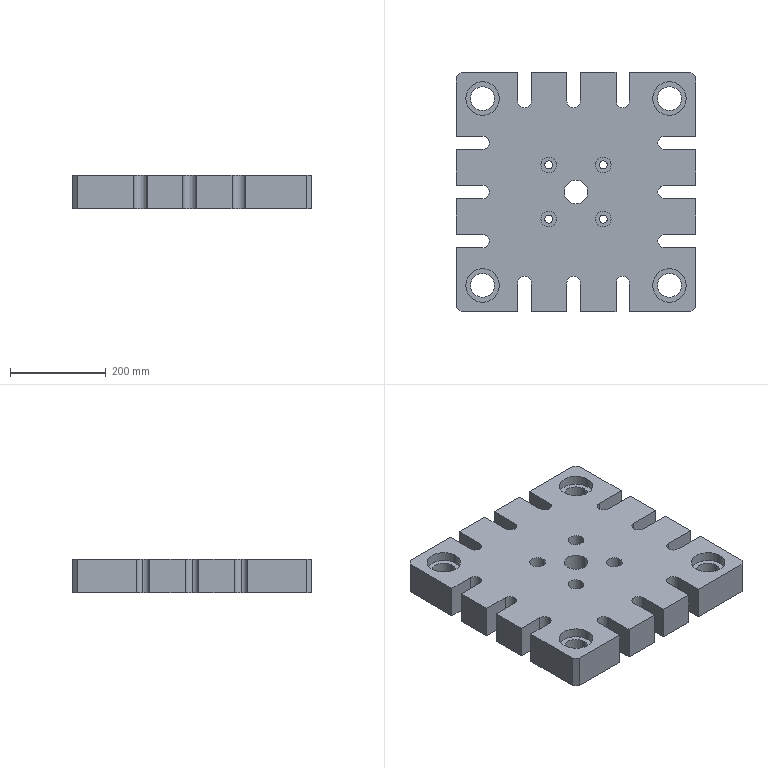Component | SolidWorks | LowerDiePlate-1 | 1 solid | 106 faces | box 500 x 500 x 70 mm | volume 14696489 mm3 | plane 55 | cylinder 51 | commonest cylinder face diameters 28 x15 50 x10 33 x8 70 x8 17 x8 200 x2
build123d program:
from build123d import *

# Parameters (mm, degrees)
SKETCH2_W               = 500
SKETCH2_H               = 500
SKETCH2_R               = 25
BOSS_EXTRUDE1_DEPTH     = 70
SKETCH3_R               = 25
CUT_EXTRUDE1_DEPTH      = 361.416
CUT_EXTRUDE2_DEPTH      = 361.416
CHAMFER1_SIZE           = 10
SKETCH5_R               = 35
CUT_EXTRUDE3_DEPTH      = 20
SKETCH6_R               = 100
CUT_EXTRUDE4_DEPTH      = 5
CUT_EXTRUDE5_DEPTH      = 360.479
CUT_EXTRUDE5_DEPTH_BACK = 360.479
SKETCH7_R               = 8.5
SKETCH8_R               = 16.5
CUT_EXTRUDE6_DEPTH      = 30


with BuildPart() as part:
    # Sketch2 → Boss-Extrude1 (new body)
    with BuildSketch(Plane.XY):
        Rectangle(SKETCH2_W, SKETCH2_H)
        Circle(SKETCH2_R, mode=Mode.SUBTRACT)
    extrude(amount=BOSS_EXTRUDE1_DEPTH)

    # Sketch3 → Cut-Extrude1 (cut, through all)
    with BuildSketch(Plane.XY.offset(70)):
        with Locations((-195, 195)):
            Circle(SKETCH3_R)
        with Locations(Location((195, 195, 0), (0, 0, 180))):
            Circle(SKETCH3_R)
        with Locations((195, -195)):
            Circle(SKETCH3_R)
        with Locations(Location((-195, -195, 0), (0, 0, 180))):
            Circle(SKETCH3_R)
    extrude(amount=-CUT_EXTRUDE1_DEPTH, mode=Mode.SUBTRACT)

    # Sketch4 → Cut-Extrude2 (cut, through all)
    with BuildSketch(Plane.XY.offset(70)):
        with BuildLine():
            Line((-195, 14), (-276.463, 14))
            Line((-276.463, 14), (-276.463, -14))
            Line((-276.463, -14), (-195, -14))
            ThreePointArc((-195, -14), (-181, 0), (-195, 14))
        make_face()
        with BuildLine():
            Line((-195, -88.5), (-276.463, -88.5))
            Line((-276.463, -88.5), (-276.463, -116.5))
            Line((-276.463, -116.5), (-195, -116.5))
            ThreePointArc((-195, -116.5), (-181, -102.5), (-195, -88.5))
        make_face()
        with BuildLine():
            Line((-276.463, 116.5), (-195, 116.5))
            ThreePointArc((-195, 116.5), (-181, 102.5), (-195, 88.5))
            Line((-195, 88.5), (-276.463, 88.5))
            Line((-276.463, 88.5), (-276.463, 116.5))
        make_face()
        with BuildLine():
            Line((83.5, 190), (83.5, 271.463))
            Line((83.5, 271.463), (111.5, 271.463))
            Line((111.5, 271.463), (111.5, 190))
            ThreePointArc((111.5, 190), (97.5, 176), (83.5, 190))
        make_face()
        with BuildLine():
            Line((9, 190), (9, 271.463))
            Line((9, 271.463), (-19, 271.463))
            Line((-19, 271.463), (-19, 190))
            ThreePointArc((-19, 190), (-5, 176), (9, 190))
        make_face()
        with BuildLine():
            Line((-93.5, 190), (-93.5, 271.463))
            Line((-93.5, 271.463), (-121.5, 271.463))
            Line((-121.5, 271.463), (-121.5, 190))
            ThreePointArc((-121.5, 190), (-107.5, 176), (-93.5, 190))
        make_face()
        with BuildLine():
            Line((185, -88.5), (266.463, -88.5))
            Line((266.463, -88.5), (266.463, -116.5))
            Line((266.463, -116.5), (185, -116.5))
            ThreePointArc((185, -116.5), (171, -102.5), (185, -88.5))
        make_face()
        with BuildLine():
            Line((185, -14), (266.463, -14))
            Line((266.463, -14), (266.463, 14))
            Line((266.463, 14), (185, 14))
            ThreePointArc((185, 14), (171, 0), (185, -14))
        make_face()
        with BuildLine():
            Line((185, 88.5), (266.463, 88.5))
            Line((266.463, 88.5), (266.463, 116.5))
            Line((266.463, 116.5), (185, 116.5))
            ThreePointArc((185, 116.5), (171, 102.5), (185, 88.5))
        make_face()
        with BuildLine():
            Line((-93.5, -190), (-93.5, -271.463))
            Line((-93.5, -271.463), (-121.5, -271.463))
            Line((-121.5, -271.463), (-121.5, -190))
            ThreePointArc((-121.5, -190), (-107.5, -176), (-93.5, -190))
        make_face()
        with BuildLine():
            Line((-19, -190), (-19, -271.463))
            Line((-19, -271.463), (9, -271.463))
            Line((9, -271.463), (9, -190))
            ThreePointArc((9, -190), (-5, -176), (-19, -190))
        make_face()
        with BuildLine():
            Line((83.5, -190), (83.5, -271.463))
            Line((83.5, -271.463), (111.5, -271.463))
            Line((111.5, -271.463), (111.5, -190))
            ThreePointArc((111.5, -190), (97.5, -176), (83.5, -190))
        make_face()
    extrude(amount=-CUT_EXTRUDE2_DEPTH, mode=Mode.SUBTRACT)

    # Chamfer1
    chamfer1_edges = [part.edges().sort_by_distance(p)[0] for p in [
        (250, -250, 35),
        (-250, -250, 35),
        (-250, 250, 35),
        (250, 250, 35),
    ]]
    chamfer(chamfer1_edges, length=CHAMFER1_SIZE)

    # Sketch5 → Cut-Extrude3 (cut)
    with BuildSketch(Plane.XY.offset(70)):
        with Locations((-195, 195)):
            Circle(SKETCH5_R)
        with Locations((195, 195)):
            Circle(SKETCH5_R)
        with Locations((195, -195)):
            Circle(SKETCH5_R)
        with Locations((-195, -195)):
            Circle(SKETCH5_R)
    extrude(amount=-CUT_EXTRUDE3_DEPTH, mode=Mode.SUBTRACT)

    # Sketch6 → Cut-Extrude4 (cut)
    with BuildSketch(Plane(origin=(0, 0, 0), x_dir=(-1, 0, 0), z_dir=(0, 0, -1))):
        Circle(SKETCH6_R)
    extrude(amount=-CUT_EXTRUDE4_DEPTH, mode=Mode.SUBTRACT)

    # Sketch7 → Cut-Extrude5 (cut, two sides: drawn at the far end of the back side and taken through both)
    with BuildSketch(Plane(origin=(0, 0, 5), x_dir=(-1, 0, 0), z_dir=(0, 0, -1)).offset(-CUT_EXTRUDE5_DEPTH_BACK)):
        with Locations((-56.569, 56.569)):
            Circle(SKETCH7_R)
        with Locations((56.569, 56.569)):
            Circle(SKETCH7_R)
        with Locations((56.569, -56.569)):
            Circle(SKETCH7_R)
        with Locations((-56.569, -56.569)):
            Circle(SKETCH7_R)
    extrude(amount=CUT_EXTRUDE5_DEPTH + CUT_EXTRUDE5_DEPTH_BACK, mode=Mode.SUBTRACT)

    # Sketch8 → Cut-Extrude6 (cut)
    with BuildSketch(Plane.XY.offset(70)):
        with Locations((-56.569, 56.569)):
            Circle(SKETCH8_R)
        with Locations((56.569, 56.569)):
            Circle(SKETCH8_R)
        with Locations((56.569, -56.569)):
            Circle(SKETCH8_R)
        with Locations((-56.569, -56.569)):
            Circle(SKETCH8_R)
    extrude(amount=-CUT_EXTRUDE6_DEPTH, mode=Mode.SUBTRACT)


solid = part.part

# Placed as in the assembly
solid = solid.moved(Location((0, 0, 75), (0, 0, 0)))